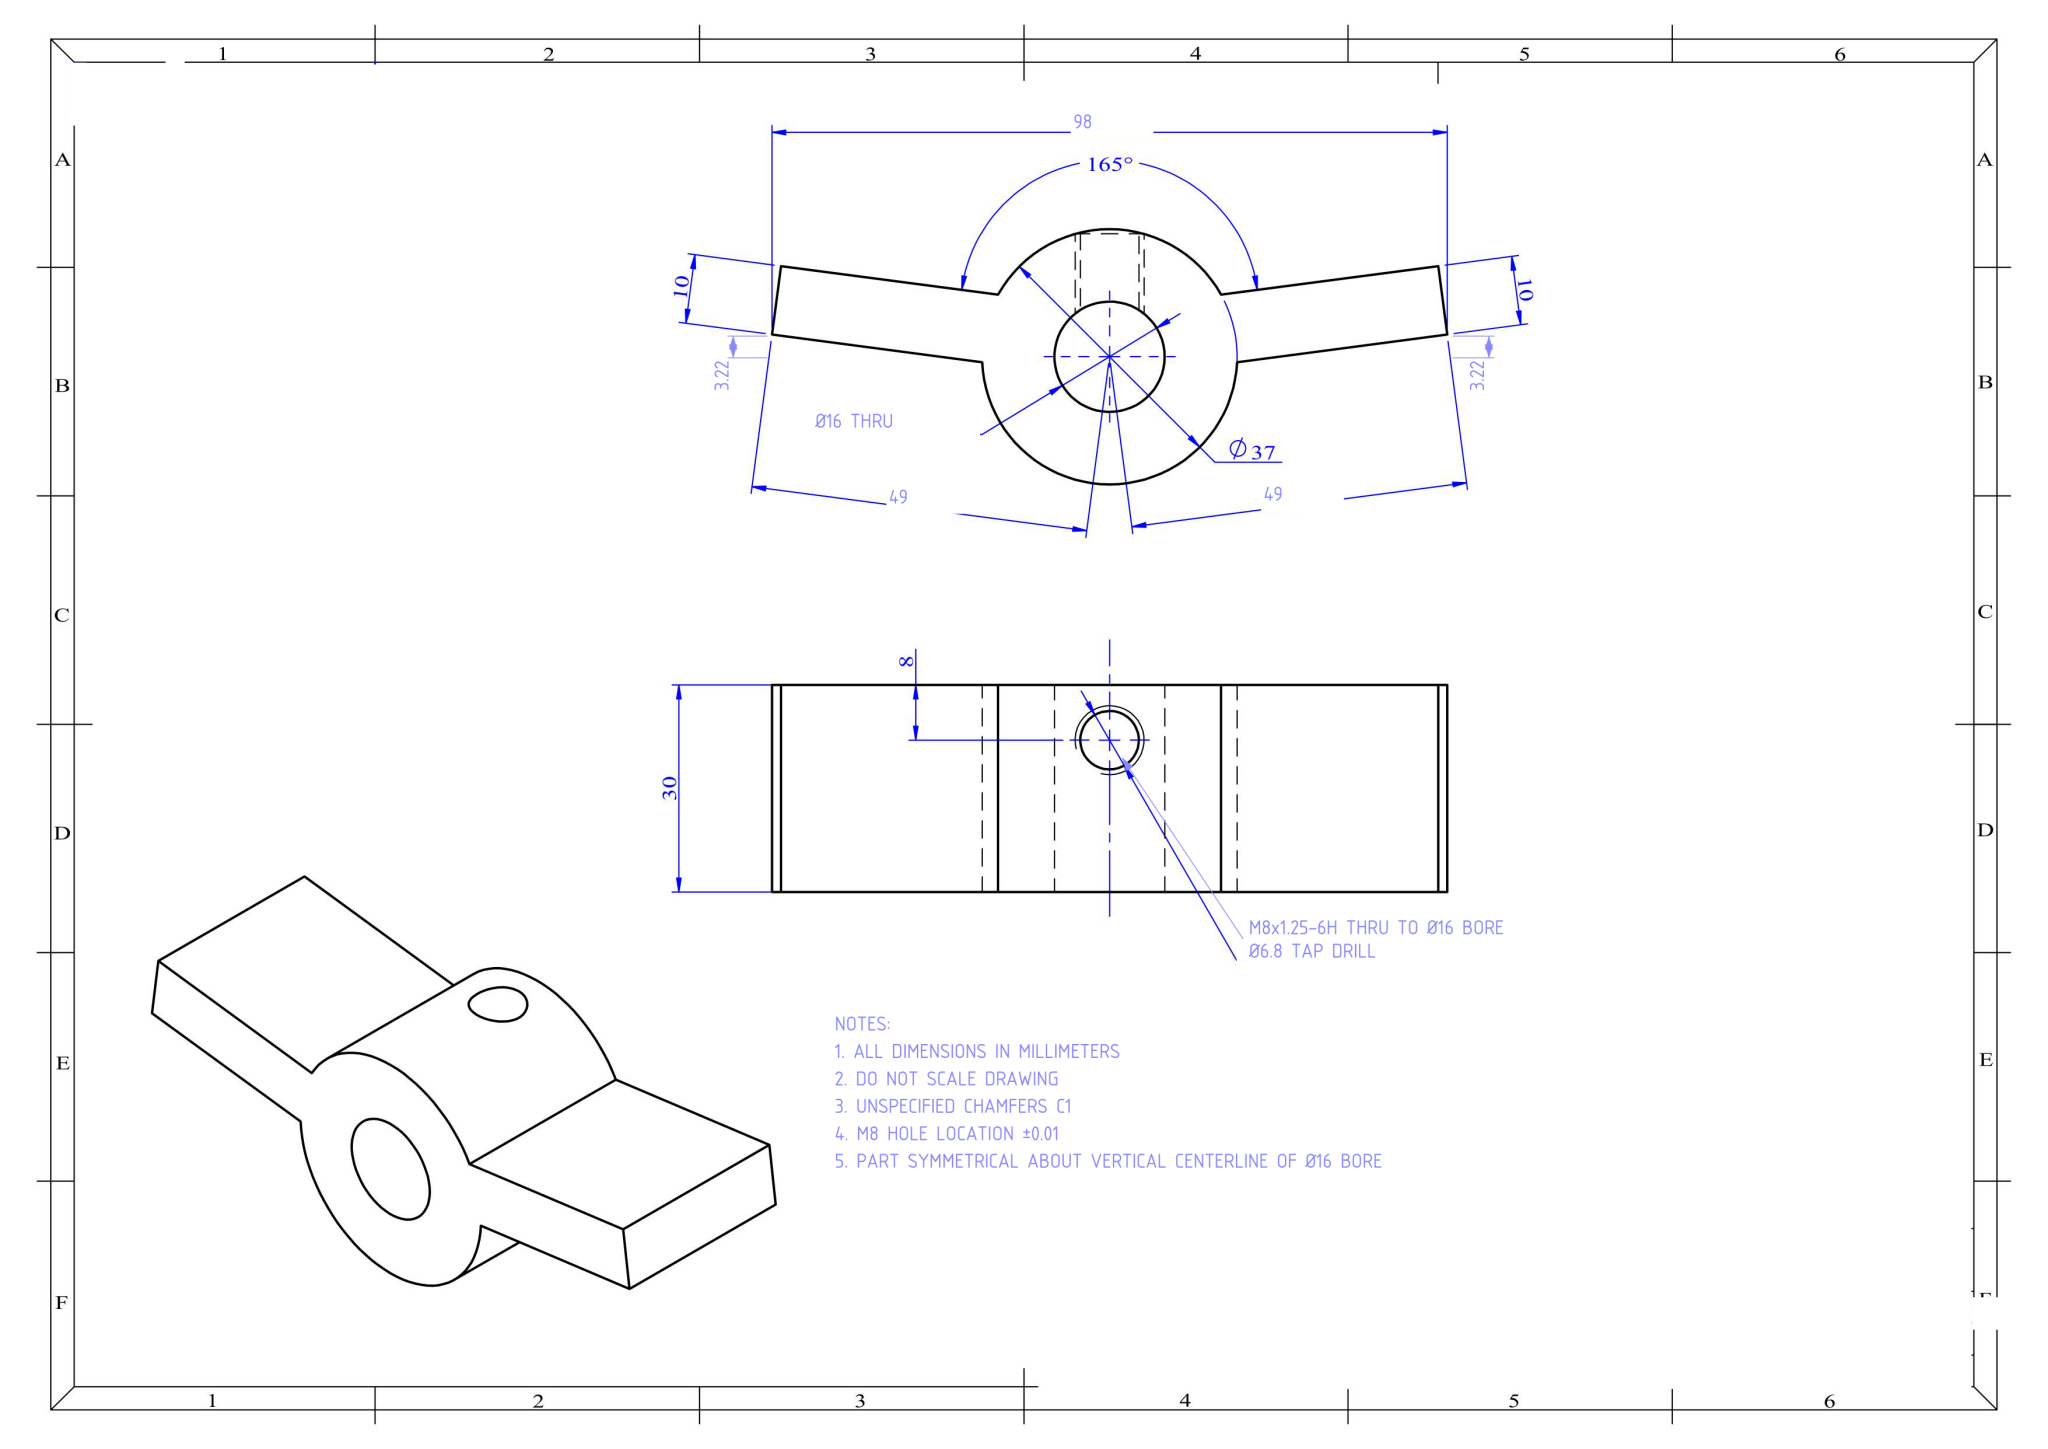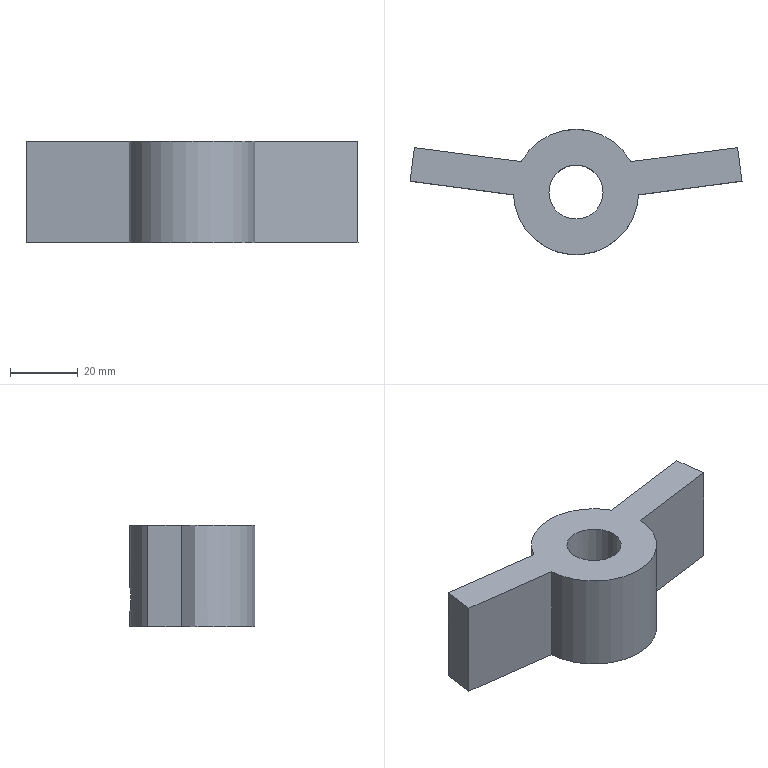Part | NX | mm | 1 solid | 14 faces | box 98 x 37 x 30 mm | volume 44321 mm3 | plane 8 | cylinder 4 | spline 2 | commonest cylinder face diameters 37 x2 16 x1 6.8 x1